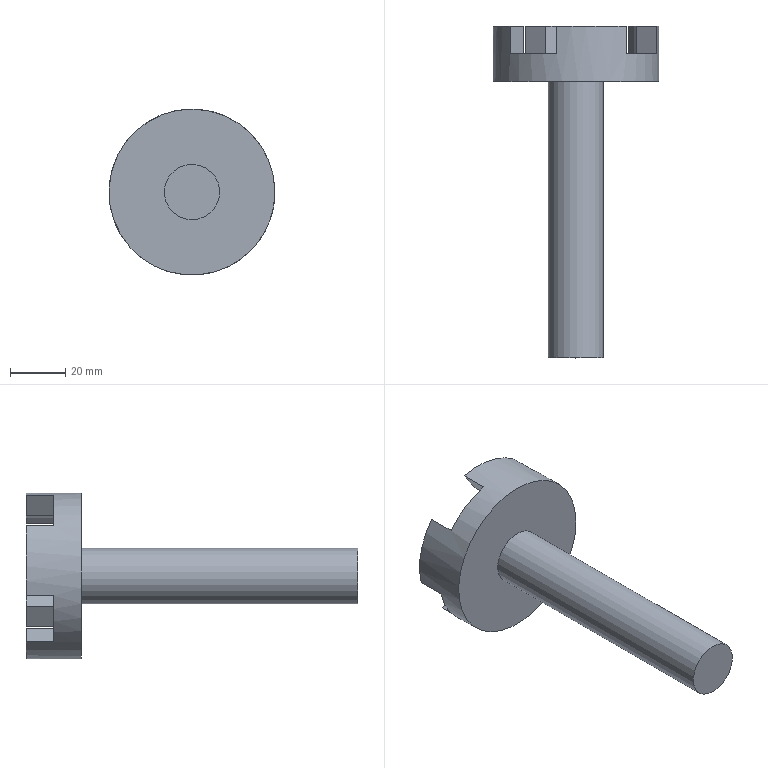Component | NX | ADJUST_SCREW_2 | 1 solid | 22 faces | volume 66209 mm3 | plane 19 | cylinder 3 | commonest cylinder face diameters 60 x1 44 x1 20 x1